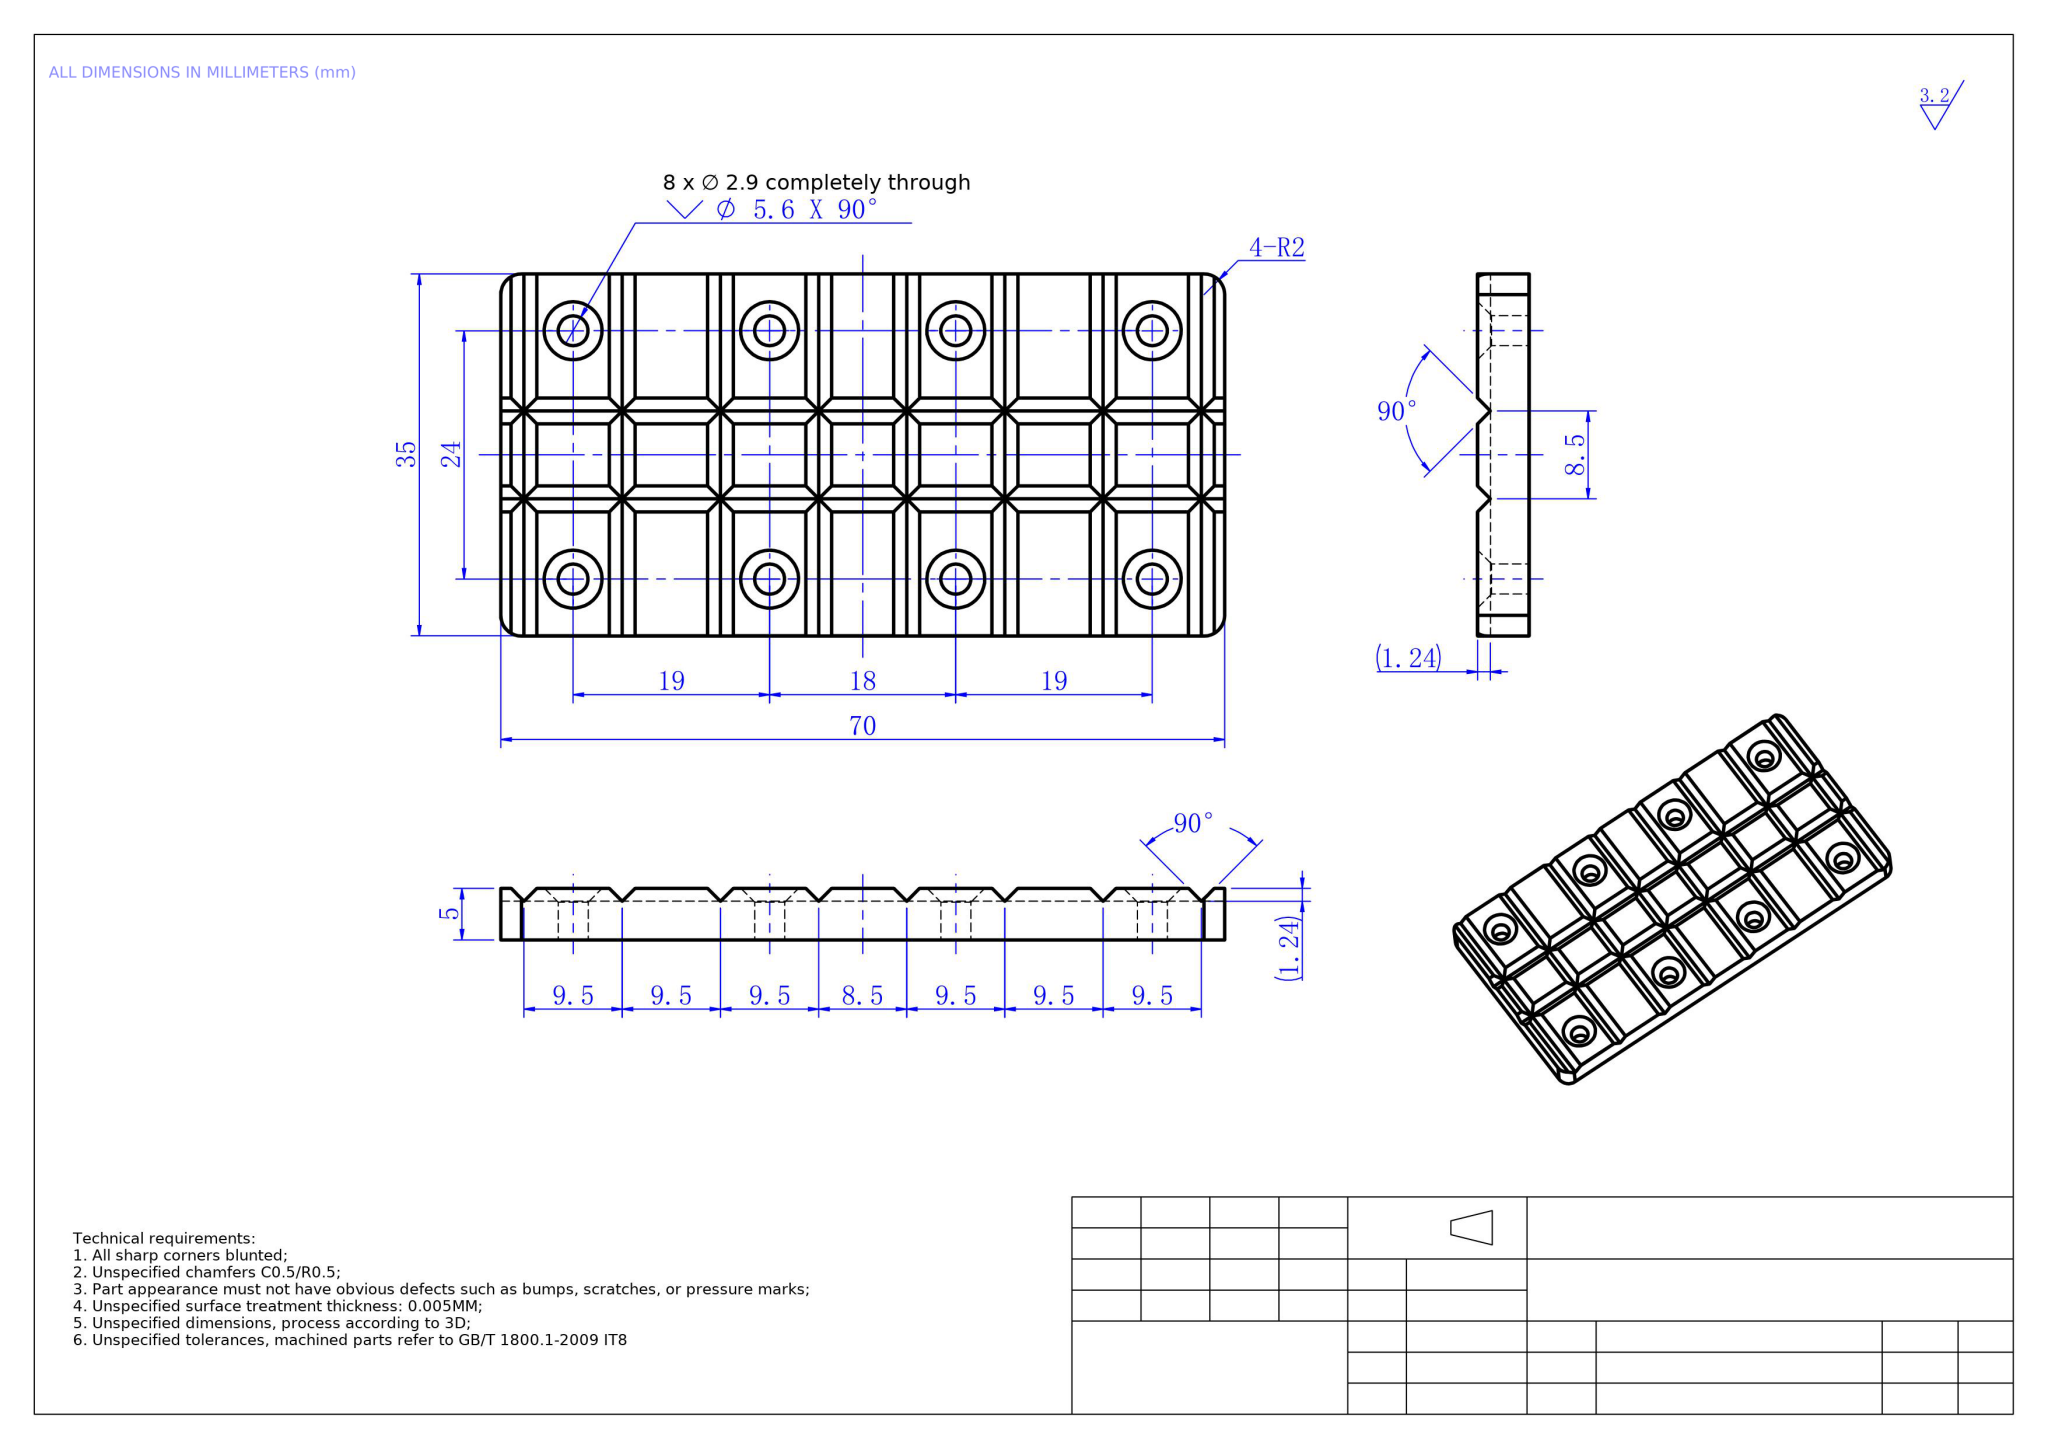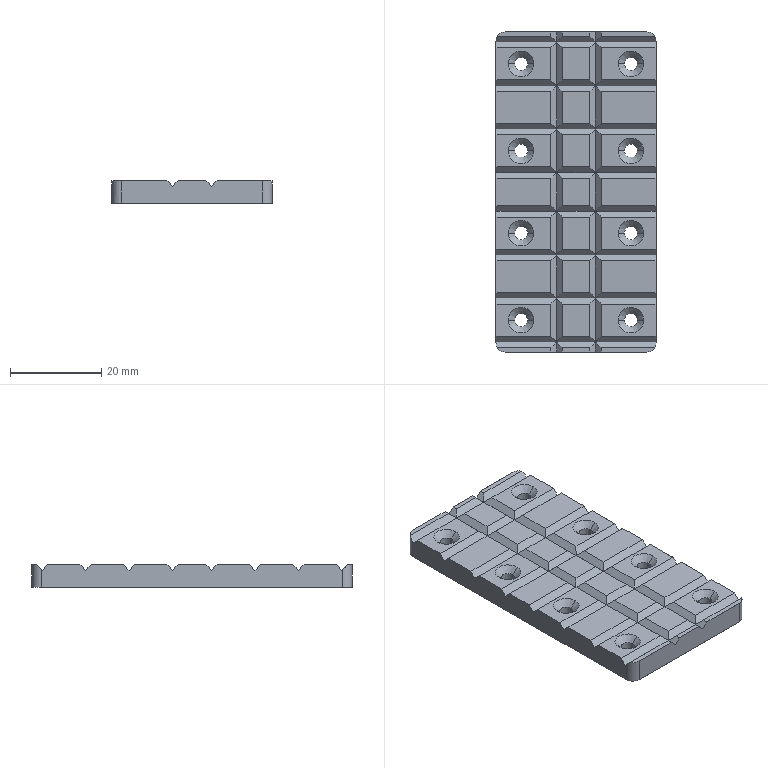Part | NX | mm | 1 solid | 184 faces | box 35 x 70 x 5 mm | volume 11267 mm3 | plane 140 | cone 24 | cylinder 20 | commonest cylinder face diameters 2.9 x16 4 x4